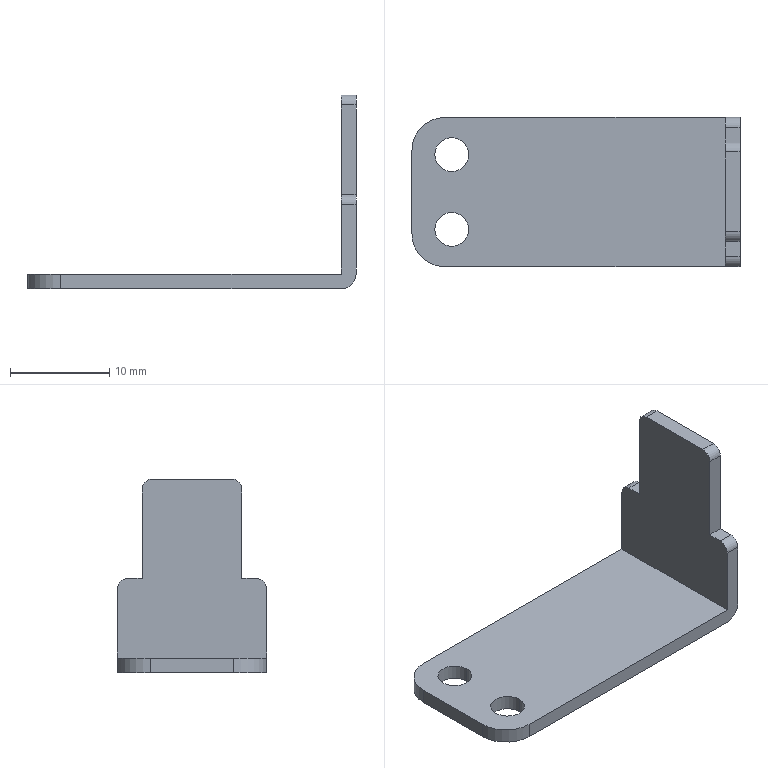Component | SolidWorks | V1ZHXTRR60SecondarySB1-1_V1ZHXT3.60InductionPlateSB1-1 | 1 solid | 23 faces | box 33 x 15 x 19.5 mm | volume 1030 mm3 | plane 12 | cylinder 11 | commonest cylinder face diameters 3.4 x4 2 x4 6.6 x2 3 x1
STEP:
#1=COLOUR_RGB('',0.7922,0.8196,0.9333);
#2=FILL_AREA_STYLE_COLOUR('',#1);
#3=FILL_AREA_STYLE('',(#2));
#4=SURFACE_STYLE_FILL_AREA(#3);
#5=SURFACE_SIDE_STYLE('',(#4));
#6=SURFACE_STYLE_USAGE(.BOTH.,#5);
#7=PRESENTATION_STYLE_ASSIGNMENT((#6));
#8=CARTESIAN_POINT('',(8.729,-7.889,17.903));
#9=VERTEX_POINT('',#8);
#10=CARTESIAN_POINT('',(8.595,-7.889,17.903));
#11=VERTEX_POINT('',#10);
#12=CARTESIAN_POINT('',(8.662,-7.889,17.903));
#13=DIRECTION('',(0.,-0.,1.));
#14=DIRECTION('',(1.,0.,0.));
#15=AXIS2_PLACEMENT_3D('',#12,#13,#14);
#16=CIRCLE('',#15,0.06693);
#17=EDGE_CURVE('',#9,#11,#16,.T.);
#18=ORIENTED_EDGE('',*,*,#17,.T.);
#19=CARTESIAN_POINT('',(8.595,-7.889,17.844));
#20=VERTEX_POINT('',#19);
#21=CARTESIAN_POINT('',(8.595,-7.889,17.844));
#22=DIRECTION('',(-0.,0.,-1.));
#23=VECTOR('',#22,39.37);
#24=LINE('',#21,#23);
#25=EDGE_CURVE('',#11,#20,#24,.T.);
#26=ORIENTED_EDGE('',*,*,#25,.T.);
#27=CARTESIAN_POINT('',(8.729,-7.889,17.844));
#28=VERTEX_POINT('',#27);
#29=CARTESIAN_POINT('',(8.662,-7.889,17.844));
#30=DIRECTION('',(0.,-0.,1.));
#31=DIRECTION('',(1.,0.,0.));
#32=AXIS2_PLACEMENT_3D('',#29,#30,#31);
#33=CIRCLE('',#32,0.06693);
#34=EDGE_CURVE('',#28,#20,#33,.T.);
#35=ORIENTED_EDGE('',*,*,#34,.F.);
#36=CARTESIAN_POINT('',(8.729,-7.889,17.844));
#37=DIRECTION('',(-0.,0.,-1.));
#38=VECTOR('',#37,39.37);
#39=LINE('',#36,#38);
#40=EDGE_CURVE('',#9,#28,#39,.T.);
#41=ORIENTED_EDGE('',*,*,#40,.F.);
#42=EDGE_LOOP('',(#18,#26,#35,#41));
#43=FACE_OUTER_BOUND('',#42,.T.);
#44=CARTESIAN_POINT('',(8.662,-7.889,17.844));
#45=DIRECTION('',(-0.,0.,-1.));
#46=DIRECTION('',(1.,0.,0.));
#47=AXIS2_PLACEMENT_3D('',#44,#45,#46);
#48=CYLINDRICAL_SURFACE('',#47,0.06693);
#49=ADVANCED_FACE('',(#43),#48,.F.);
#50=CARTESIAN_POINT('',(8.729,-8.184,17.903));
#51=VERTEX_POINT('',#50);
#52=CARTESIAN_POINT('',(8.595,-8.184,17.903));
#53=VERTEX_POINT('',#52);
#54=CARTESIAN_POINT('',(8.662,-8.184,17.903));
#55=DIRECTION('',(0.,-0.,1.));
#56=DIRECTION('',(1.,0.,0.));
#57=AXIS2_PLACEMENT_3D('',#54,#55,#56);
#58=CIRCLE('',#57,0.06693);
#59=EDGE_CURVE('',#51,#53,#58,.T.);
#60=ORIENTED_EDGE('',*,*,#59,.T.);
#61=CARTESIAN_POINT('',(8.595,-8.184,17.844));
#62=VERTEX_POINT('',#61);
#63=CARTESIAN_POINT('',(8.595,-8.184,17.844));
#64=DIRECTION('',(-0.,0.,-1.));
#65=VECTOR('',#64,39.37);
#66=LINE('',#63,#65);
#67=EDGE_CURVE('',#53,#62,#66,.T.);
#68=ORIENTED_EDGE('',*,*,#67,.T.);
#69=CARTESIAN_POINT('',(8.729,-8.184,17.844));
#70=VERTEX_POINT('',#69);
#71=CARTESIAN_POINT('',(8.662,-8.184,17.844));
#72=DIRECTION('',(0.,-0.,1.));
#73=DIRECTION('',(1.,0.,0.));
#74=AXIS2_PLACEMENT_3D('',#71,#72,#73);
#75=CIRCLE('',#74,0.06693);
#76=EDGE_CURVE('',#70,#62,#75,.T.);
#77=ORIENTED_EDGE('',*,*,#76,.F.);
#78=CARTESIAN_POINT('',(8.729,-8.184,17.844));
#79=DIRECTION('',(-0.,0.,-1.));
#80=VECTOR('',#79,39.37);
#81=LINE('',#78,#80);
#82=EDGE_CURVE('',#51,#70,#81,.T.);
#83=ORIENTED_EDGE('',*,*,#82,.F.);
#84=EDGE_LOOP('',(#60,#68,#77,#83));
#85=FACE_OUTER_BOUND('',#84,.T.);
#86=CARTESIAN_POINT('',(8.662,-8.184,17.844));
#87=DIRECTION('',(-0.,0.,-1.));
#88=DIRECTION('',(1.,0.,0.));
#89=AXIS2_PLACEMENT_3D('',#86,#87,#88);
#90=CYLINDRICAL_SURFACE('',#89,0.06693);
#91=ADVANCED_FACE('',(#85),#90,.F.);
#92=CARTESIAN_POINT('',(8.505,-7.871,17.903));
#93=VERTEX_POINT('',#92);
#94=CARTESIAN_POINT('',(8.635,-7.741,17.903));
#95=VERTEX_POINT('',#94);
#96=CARTESIAN_POINT('',(8.635,-7.871,17.903));
#97=DIRECTION('',(-0.,0.,-1.));
#98=DIRECTION('',(1.,0.,0.));
#99=AXIS2_PLACEMENT_3D('',#96,#97,#98);
#100=CIRCLE('',#99,0.1299);
#101=EDGE_CURVE('',#93,#95,#100,.T.);
#102=ORIENTED_EDGE('',*,*,#101,.F.);
#103=CARTESIAN_POINT('',(8.505,-8.202,17.903));
#104=VERTEX_POINT('',#103);
#105=CARTESIAN_POINT('',(8.505,-8.332,17.903));
#106=DIRECTION('',(-0.,1.,0.));
#107=VECTOR('',#106,39.37);
#108=LINE('',#105,#107);
#109=EDGE_CURVE('',#104,#93,#108,.T.);
#110=ORIENTED_EDGE('',*,*,#109,.F.);
#111=CARTESIAN_POINT('',(8.635,-8.332,17.903));
#112=VERTEX_POINT('',#111);
#113=CARTESIAN_POINT('',(8.635,-8.202,17.903));
#114=DIRECTION('',(-0.,0.,-1.));
#115=DIRECTION('',(1.,0.,0.));
#116=AXIS2_PLACEMENT_3D('',#113,#114,#115);
#117=CIRCLE('',#116,0.1299);
#118=EDGE_CURVE('',#112,#104,#117,.T.);
#119=ORIENTED_EDGE('',*,*,#118,.F.);
#120=CARTESIAN_POINT('',(9.745,-8.332,17.903));
#121=VERTEX_POINT('',#120);
#122=CARTESIAN_POINT('',(9.804,-8.332,17.903));
#123=DIRECTION('',(-1.,-0.,0.));
#124=VECTOR('',#123,39.37);
#125=LINE('',#122,#124);
#126=EDGE_CURVE('',#121,#112,#125,.T.);
#127=ORIENTED_EDGE('',*,*,#126,.F.);
#128=CARTESIAN_POINT('',(9.745,-7.741,17.903));
#129=VERTEX_POINT('',#128);
#130=CARTESIAN_POINT('',(9.745,-8.332,17.903));
#131=DIRECTION('',(0.,-1.,-0.));
#132=VECTOR('',#131,39.37);
#133=LINE('',#130,#132);
#134=EDGE_CURVE('',#129,#121,#133,.T.);
#135=ORIENTED_EDGE('',*,*,#134,.F.);
#136=CARTESIAN_POINT('',(9.804,-7.741,17.903));
#137=DIRECTION('',(1.,0.,-0.));
#138=VECTOR('',#137,39.37);
#139=LINE('',#136,#138);
#140=EDGE_CURVE('',#95,#129,#139,.T.);
#141=ORIENTED_EDGE('',*,*,#140,.F.);
#142=EDGE_LOOP('',(#102,#110,#119,#127,#135,#141));
#143=FACE_OUTER_BOUND('',#142,.T.);
#144=ORIENTED_EDGE('',*,*,#17,.F.);
#145=CARTESIAN_POINT('',(8.662,-7.889,17.903));
#146=DIRECTION('',(0.,-0.,1.));
#147=DIRECTION('',(1.,0.,0.));
#148=AXIS2_PLACEMENT_3D('',#145,#146,#147);
#149=CIRCLE('',#148,0.06693);
#150=EDGE_CURVE('',#11,#9,#149,.T.);
#151=ORIENTED_EDGE('',*,*,#150,.F.);
#152=EDGE_LOOP('',(#144,#151));
#153=FACE_BOUND('',#152,.T.);
#154=ORIENTED_EDGE('',*,*,#59,.F.);
#155=CARTESIAN_POINT('',(8.662,-8.184,17.903));
#156=DIRECTION('',(0.,-0.,1.));
#157=DIRECTION('',(1.,0.,0.));
#158=AXIS2_PLACEMENT_3D('',#155,#156,#157);
#159=CIRCLE('',#158,0.06693);
#160=EDGE_CURVE('',#53,#51,#159,.T.);
#161=ORIENTED_EDGE('',*,*,#160,.F.);
#162=EDGE_LOOP('',(#154,#161));
#163=FACE_BOUND('',#162,.T.);
#164=CARTESIAN_POINT('',(9.804,-8.332,17.903));
#165=DIRECTION('',(-0.,0.,-1.));
#166=DIRECTION('',(1.,0.,-0.));
#167=AXIS2_PLACEMENT_3D('',#164,#165,#166);
#168=PLANE('',#167);
#169=ADVANCED_FACE('',(#143,#153,#163),#168,.F.);
#170=CARTESIAN_POINT('',(9.745,-7.741,17.844));
#171=VERTEX_POINT('',#170);
#172=CARTESIAN_POINT('',(9.804,-7.741,17.903));
#173=VERTEX_POINT('',#172);
#174=CARTESIAN_POINT('',(9.745,-7.741,17.903));
#175=DIRECTION('',(0.,-1.,-0.));
#176=DIRECTION('',(0.,-0.,1.));
#177=AXIS2_PLACEMENT_3D('',#174,#175,#176);
#178=CIRCLE('',#177,0.05906);
#179=EDGE_CURVE('',#171,#173,#178,.T.);
#180=ORIENTED_EDGE('',*,*,#179,.F.);
#181=CARTESIAN_POINT('',(8.635,-7.741,17.844));
#182=VERTEX_POINT('',#181);
#183=CARTESIAN_POINT('',(9.804,-7.741,17.844));
#184=DIRECTION('',(1.,0.,-0.));
#185=VECTOR('',#184,39.37);
#186=LINE('',#183,#185);
#187=EDGE_CURVE('',#182,#171,#186,.T.);
#188=ORIENTED_EDGE('',*,*,#187,.F.);
#189=CARTESIAN_POINT('',(8.635,-7.741,17.903));
#190=DIRECTION('',(-0.,0.,-1.));
#191=VECTOR('',#190,39.37);
#192=LINE('',#189,#191);
#193=EDGE_CURVE('',#95,#182,#192,.T.);
#194=ORIENTED_EDGE('',*,*,#193,.F.);
#195=ORIENTED_EDGE('',*,*,#140,.T.);
#196=CARTESIAN_POINT('',(9.745,-7.741,18.179));
#197=VERTEX_POINT('',#196);
#198=CARTESIAN_POINT('',(9.745,-7.741,17.903));
#199=DIRECTION('',(-0.,0.,-1.));
#200=VECTOR('',#199,39.37);
#201=LINE('',#198,#200);
#202=EDGE_CURVE('',#197,#129,#201,.T.);
#203=ORIENTED_EDGE('',*,*,#202,.F.);
#204=CARTESIAN_POINT('',(9.804,-7.741,18.179));
#205=VERTEX_POINT('',#204);
#206=CARTESIAN_POINT('',(9.804,-7.741,18.179));
#207=DIRECTION('',(-1.,-0.,0.));
#208=VECTOR('',#207,39.37);
#209=LINE('',#206,#208);
#210=EDGE_CURVE('',#205,#197,#209,.T.);
#211=ORIENTED_EDGE('',*,*,#210,.F.);
#212=CARTESIAN_POINT('',(9.804,-7.741,17.903));
#213=DIRECTION('',(0.,-0.,1.));
#214=VECTOR('',#213,39.37);
#215=LINE('',#212,#214);
#216=EDGE_CURVE('',#173,#205,#215,.T.);
#217=ORIENTED_EDGE('',*,*,#216,.F.);
#218=EDGE_LOOP('',(#180,#188,#194,#195,#203,#211,#217));
#219=FACE_OUTER_BOUND('',#218,.T.);
#220=CARTESIAN_POINT('',(9.804,-7.741,17.903));
#221=DIRECTION('',(0.,-1.,-0.));
#222=DIRECTION('',(0.,-0.,1.));
#223=AXIS2_PLACEMENT_3D('',#220,#221,#222);
#224=PLANE('',#223);
#225=ADVANCED_FACE('',(#219),#224,.F.);
#226=CARTESIAN_POINT('',(8.505,-7.871,17.844));
#227=VERTEX_POINT('',#226);
#228=CARTESIAN_POINT('',(8.635,-7.871,17.844));
#229=DIRECTION('',(0.,-0.,1.));
#230=DIRECTION('',(1.,0.,0.));
#231=AXIS2_PLACEMENT_3D('',#228,#229,#230);
#232=CIRCLE('',#231,0.1299);
#233=EDGE_CURVE('',#182,#227,#232,.T.);
#234=ORIENTED_EDGE('',*,*,#233,.T.);
#235=CARTESIAN_POINT('',(8.505,-7.871,17.903));
#236=DIRECTION('',(0.,-0.,1.));
#237=VECTOR('',#236,39.37);
#238=LINE('',#235,#237);
#239=EDGE_CURVE('',#227,#93,#238,.T.);
#240=ORIENTED_EDGE('',*,*,#239,.T.);
#241=ORIENTED_EDGE('',*,*,#101,.T.);
#242=ORIENTED_EDGE('',*,*,#193,.T.);
#243=EDGE_LOOP('',(#234,#240,#241,#242));
#244=FACE_OUTER_BOUND('',#243,.T.);
#245=CARTESIAN_POINT('',(8.635,-7.871,17.903));
#246=DIRECTION('',(-0.,0.,-1.));
#247=DIRECTION('',(1.,0.,0.));
#248=AXIS2_PLACEMENT_3D('',#245,#246,#247);
#249=CYLINDRICAL_SURFACE('',#248,0.1299);
#250=ADVANCED_FACE('',(#244),#249,.T.);
#251=ORIENTED_EDGE('',*,*,#239,.F.);
#252=CARTESIAN_POINT('',(8.505,-8.202,17.844));
#253=VERTEX_POINT('',#252);
#254=CARTESIAN_POINT('',(8.505,-7.741,17.844));
#255=DIRECTION('',(-0.,1.,0.));
#256=VECTOR('',#255,39.37);
#257=LINE('',#254,#256);
#258=EDGE_CURVE('',#253,#227,#257,.T.);
#259=ORIENTED_EDGE('',*,*,#258,.F.);
#260=CARTESIAN_POINT('',(8.505,-8.202,17.903));
#261=DIRECTION('',(-0.,0.,-1.));
#262=VECTOR('',#261,39.37);
#263=LINE('',#260,#262);
#264=EDGE_CURVE('',#104,#253,#263,.T.);
#265=ORIENTED_EDGE('',*,*,#264,.F.);
#266=ORIENTED_EDGE('',*,*,#109,.T.);
#267=EDGE_LOOP('',(#251,#259,#265,#266));
#268=FACE_OUTER_BOUND('',#267,.T.);
#269=CARTESIAN_POINT('',(8.505,-7.741,17.903));
#270=DIRECTION('',(1.,0.,-0.));
#271=DIRECTION('',(0.,-0.,1.));
#272=AXIS2_PLACEMENT_3D('',#269,#270,#271);
#273=PLANE('',#272);
#274=ADVANCED_FACE('',(#268),#273,.F.);
#275=CARTESIAN_POINT('',(8.635,-8.332,17.844));
#276=VERTEX_POINT('',#275);
#277=CARTESIAN_POINT('',(8.635,-8.202,17.844));
#278=DIRECTION('',(0.,-0.,1.));
#279=DIRECTION('',(1.,0.,0.));
#280=AXIS2_PLACEMENT_3D('',#277,#278,#279);
#281=CIRCLE('',#280,0.1299);
#282=EDGE_CURVE('',#253,#276,#281,.T.);
#283=ORIENTED_EDGE('',*,*,#282,.T.);
#284=CARTESIAN_POINT('',(8.635,-8.332,17.903));
#285=DIRECTION('',(0.,-0.,1.));
#286=VECTOR('',#285,39.37);
#287=LINE('',#284,#286);
#288=EDGE_CURVE('',#276,#112,#287,.T.);
#289=ORIENTED_EDGE('',*,*,#288,.T.);
#290=ORIENTED_EDGE('',*,*,#118,.T.);
#291=ORIENTED_EDGE('',*,*,#264,.T.);
#292=EDGE_LOOP('',(#283,#289,#290,#291));
#293=FACE_OUTER_BOUND('',#292,.T.);
#294=CARTESIAN_POINT('',(8.635,-8.202,17.903));
#295=DIRECTION('',(-0.,0.,-1.));
#296=DIRECTION('',(1.,0.,0.));
#297=AXIS2_PLACEMENT_3D('',#294,#295,#296);
#298=CYLINDRICAL_SURFACE('',#297,0.1299);
#299=ADVANCED_FACE('',(#293),#298,.T.);
#300=CARTESIAN_POINT('',(9.804,-8.332,17.903));
#301=VERTEX_POINT('',#300);
#302=CARTESIAN_POINT('',(9.745,-8.332,17.844));
#303=VERTEX_POINT('',#302);
#304=CARTESIAN_POINT('',(9.745,-8.332,17.903));
#305=DIRECTION('',(-0.,1.,0.));
#306=DIRECTION('',(0.,-0.,1.));
#307=AXIS2_PLACEMENT_3D('',#304,#305,#306);
#308=CIRCLE('',#307,0.05906);
#309=EDGE_CURVE('',#301,#303,#308,.T.);
#310=ORIENTED_EDGE('',*,*,#309,.F.);
#311=CARTESIAN_POINT('',(9.804,-8.332,18.179));
#312=VERTEX_POINT('',#311);
#313=CARTESIAN_POINT('',(9.804,-8.332,17.903));
#314=DIRECTION('',(-0.,0.,-1.));
#315=VECTOR('',#314,39.37);
#316=LINE('',#313,#315);
#317=EDGE_CURVE('',#312,#301,#316,.T.);
#318=ORIENTED_EDGE('',*,*,#317,.F.);
#319=CARTESIAN_POINT('',(9.745,-8.332,18.179));
#320=VERTEX_POINT('',#319);
#321=CARTESIAN_POINT('',(9.804,-8.332,18.179));
#322=DIRECTION('',(1.,0.,-0.));
#323=VECTOR('',#322,39.37);
#324=LINE('',#321,#323);
#325=EDGE_CURVE('',#320,#312,#324,.T.);
#326=ORIENTED_EDGE('',*,*,#325,.F.);
#327=CARTESIAN_POINT('',(9.745,-8.332,17.903));
#328=DIRECTION('',(0.,-0.,1.));
#329=VECTOR('',#328,39.37);
#330=LINE('',#327,#329);
#331=EDGE_CURVE('',#121,#320,#330,.T.);
#332=ORIENTED_EDGE('',*,*,#331,.F.);
#333=ORIENTED_EDGE('',*,*,#126,.T.);
#334=ORIENTED_EDGE('',*,*,#288,.F.);
#335=CARTESIAN_POINT('',(9.804,-8.332,17.844));
#336=DIRECTION('',(-1.,-0.,0.));
#337=VECTOR('',#336,39.37);
#338=LINE('',#335,#337);
#339=EDGE_CURVE('',#303,#276,#338,.T.);
#340=ORIENTED_EDGE('',*,*,#339,.F.);
#341=EDGE_LOOP('',(#310,#318,#326,#332,#333,#334,#340));
#342=FACE_OUTER_BOUND('',#341,.T.);
#343=CARTESIAN_POINT('',(9.804,-8.332,17.903));
#344=DIRECTION('',(-0.,1.,0.));
#345=DIRECTION('',(-0.,0.,-1.));
#346=AXIS2_PLACEMENT_3D('',#343,#344,#345);
#347=PLANE('',#346);
#348=ADVANCED_FACE('',(#342),#347,.F.);
#349=CARTESIAN_POINT('',(9.745,-8.293,18.218));
#350=VERTEX_POINT('',#349);
#351=CARTESIAN_POINT('',(9.745,-8.293,18.179));
#352=DIRECTION('',(1.,0.,-0.));
#353=DIRECTION('',(0.,-0.,1.));
#354=AXIS2_PLACEMENT_3D('',#351,#352,#353);
#355=CIRCLE('',#354,0.03937);
#356=EDGE_CURVE('',#350,#320,#355,.T.);
#357=ORIENTED_EDGE('',*,*,#356,.F.);
#358=CARTESIAN_POINT('',(9.745,-8.234,18.218));
#359=VERTEX_POINT('',#358);
#360=CARTESIAN_POINT('',(9.745,-8.332,18.218));
#361=DIRECTION('',(0.,-1.,-0.));
#362=VECTOR('',#361,39.37);
#363=LINE('',#360,#362);
#364=EDGE_CURVE('',#359,#350,#363,.T.);
#365=ORIENTED_EDGE('',*,*,#364,.F.);
#366=CARTESIAN_POINT('',(9.745,-8.234,18.572));
#367=VERTEX_POINT('',#366);
#368=CARTESIAN_POINT('',(9.745,-8.234,18.612));
#369=DIRECTION('',(-0.,0.,-1.));
#370=VECTOR('',#369,39.37);
#371=LINE('',#368,#370);
#372=EDGE_CURVE('',#367,#359,#371,.T.);
#373=ORIENTED_EDGE('',*,*,#372,.F.);
#374=CARTESIAN_POINT('',(9.745,-8.194,18.612));
#375=VERTEX_POINT('',#374);
#376=CARTESIAN_POINT('',(9.745,-8.194,18.572));
#377=DIRECTION('',(1.,0.,-0.));
#378=DIRECTION('',(0.,-0.,1.));
#379=AXIS2_PLACEMENT_3D('',#376,#377,#378);
#380=CIRCLE('',#379,0.03937);
#381=EDGE_CURVE('',#375,#367,#380,.T.);
#382=ORIENTED_EDGE('',*,*,#381,.F.);
#383=CARTESIAN_POINT('',(9.745,-7.879,18.612));
#384=VERTEX_POINT('',#383);
#385=CARTESIAN_POINT('',(9.745,-8.332,18.612));
#386=DIRECTION('',(0.,-1.,-0.));
#387=VECTOR('',#386,39.37);
#388=LINE('',#385,#387);
#389=EDGE_CURVE('',#384,#375,#388,.T.);
#390=ORIENTED_EDGE('',*,*,#389,.F.);
#391=CARTESIAN_POINT('',(9.745,-7.84,18.572));
#392=VERTEX_POINT('',#391);
#393=CARTESIAN_POINT('',(9.745,-7.879,18.572));
#394=DIRECTION('',(1.,0.,-0.));
#395=DIRECTION('',(0.,0.,-1.));
#396=AXIS2_PLACEMENT_3D('',#393,#394,#395);
#397=CIRCLE('',#396,0.03937);
#398=EDGE_CURVE('',#392,#384,#397,.T.);
#399=ORIENTED_EDGE('',*,*,#398,.F.);
#400=CARTESIAN_POINT('',(9.745,-7.84,18.218));
#401=VERTEX_POINT('',#400);
#402=CARTESIAN_POINT('',(9.745,-7.84,18.612));
#403=DIRECTION('',(0.,-0.,1.));
#404=VECTOR('',#403,39.37);
#405=LINE('',#402,#404);
#406=EDGE_CURVE('',#401,#392,#405,.T.);
#407=ORIENTED_EDGE('',*,*,#406,.F.);
#408=CARTESIAN_POINT('',(9.745,-7.781,18.218));
#409=VERTEX_POINT('',#408);
#410=CARTESIAN_POINT('',(9.745,-8.332,18.218));
#411=DIRECTION('',(0.,-1.,-0.));
#412=VECTOR('',#411,39.37);
#413=LINE('',#410,#412);
#414=EDGE_CURVE('',#409,#401,#413,.T.);
#415=ORIENTED_EDGE('',*,*,#414,.F.);
#416=CARTESIAN_POINT('',(9.745,-7.781,18.179));
#417=DIRECTION('',(1.,0.,-0.));
#418=DIRECTION('',(0.,-0.,1.));
#419=AXIS2_PLACEMENT_3D('',#416,#417,#418);
#420=CIRCLE('',#419,0.03937);
#421=EDGE_CURVE('',#197,#409,#420,.T.);
#422=ORIENTED_EDGE('',*,*,#421,.F.);
#423=ORIENTED_EDGE('',*,*,#202,.T.);
#424=ORIENTED_EDGE('',*,*,#134,.T.);
#425=ORIENTED_EDGE('',*,*,#331,.T.);
#426=EDGE_LOOP('',(#357,#365,#373,#382,#390,#399,#407,#415,#422,#423,#424,#425));
#427=FACE_OUTER_BOUND('',#426,.T.);
#428=CARTESIAN_POINT('',(9.745,-8.332,18.612));
#429=DIRECTION('',(1.,0.,-0.));
#430=DIRECTION('',(-0.,1.,0.));
#431=AXIS2_PLACEMENT_3D('',#428,#429,#430);
#432=PLANE('',#431);
#433=ADVANCED_FACE('',(#427),#432,.F.);
#434=ORIENTED_EDGE('',*,*,#25,.F.);
#435=ORIENTED_EDGE('',*,*,#150,.T.);
#436=ORIENTED_EDGE('',*,*,#40,.T.);
#437=CARTESIAN_POINT('',(8.662,-7.889,17.844));
#438=DIRECTION('',(0.,-0.,1.));
#439=DIRECTION('',(1.,0.,0.));
#440=AXIS2_PLACEMENT_3D('',#437,#438,#439);
#441=CIRCLE('',#440,0.06693);
#442=EDGE_CURVE('',#20,#28,#441,.T.);
#443=ORIENTED_EDGE('',*,*,#442,.F.);
#444=EDGE_LOOP('',(#434,#435,#436,#443));
#445=FACE_OUTER_BOUND('',#444,.T.);
#446=CARTESIAN_POINT('',(8.662,-7.889,17.844));
#447=DIRECTION('',(-0.,0.,-1.));
#448=DIRECTION('',(1.,0.,0.));
#449=AXIS2_PLACEMENT_3D('',#446,#447,#448);
#450=CYLINDRICAL_SURFACE('',#449,0.06693);
#451=ADVANCED_FACE('',(#445),#450,.F.);
#452=ORIENTED_EDGE('',*,*,#67,.F.);
#453=ORIENTED_EDGE('',*,*,#160,.T.);
#454=ORIENTED_EDGE('',*,*,#82,.T.);
#455=CARTESIAN_POINT('',(8.662,-8.184,17.844));
#456=DIRECTION('',(0.,-0.,1.));
#457=DIRECTION('',(1.,0.,0.));
#458=AXIS2_PLACEMENT_3D('',#455,#456,#457);
#459=CIRCLE('',#458,0.06693);
#460=EDGE_CURVE('',#62,#70,#459,.T.);
#461=ORIENTED_EDGE('',*,*,#460,.F.);
#462=EDGE_LOOP('',(#452,#453,#454,#461));
#463=FACE_OUTER_BOUND('',#462,.T.);
#464=CARTESIAN_POINT('',(8.662,-8.184,17.844));
#465=DIRECTION('',(-0.,0.,-1.));
#466=DIRECTION('',(1.,0.,0.));
#467=AXIS2_PLACEMENT_3D('',#464,#465,#466);
#468=CYLINDRICAL_SURFACE('',#467,0.06693);
#469=ADVANCED_FACE('',(#463),#468,.F.);
#470=CARTESIAN_POINT('',(9.804,-7.741,17.903));
#471=DIRECTION('',(0.,-1.,-0.));
#472=VECTOR('',#471,39.37);
#473=LINE('',#470,#472);
#474=EDGE_CURVE('',#173,#301,#473,.T.);
#475=ORIENTED_EDGE('',*,*,#474,.F.);
#476=ORIENTED_EDGE('',*,*,#216,.T.);
#477=CARTESIAN_POINT('',(9.804,-7.781,18.218));
#478=VERTEX_POINT('',#477);
#479=CARTESIAN_POINT('',(9.804,-7.781,18.179));
#480=DIRECTION('',(-1.,-0.,0.));
#481=DIRECTION('',(0.,-0.,1.));
#482=AXIS2_PLACEMENT_3D('',#479,#480,#481);
#483=CIRCLE('',#482,0.03937);
#484=EDGE_CURVE('',#478,#205,#483,.T.);
#485=ORIENTED_EDGE('',*,*,#484,.F.);
#486=CARTESIAN_POINT('',(9.804,-7.84,18.218));
#487=VERTEX_POINT('',#486);
#488=CARTESIAN_POINT('',(9.804,-7.741,18.218));
#489=DIRECTION('',(-0.,1.,0.));
#490=VECTOR('',#489,39.37);
#491=LINE('',#488,#490);
#492=EDGE_CURVE('',#487,#478,#491,.T.);
#493=ORIENTED_EDGE('',*,*,#492,.F.);
#494=CARTESIAN_POINT('',(9.804,-7.84,18.572));
#495=VERTEX_POINT('',#494);
#496=CARTESIAN_POINT('',(9.804,-7.84,17.903));
#497=DIRECTION('',(-0.,0.,-1.));
#498=VECTOR('',#497,39.37);
#499=LINE('',#496,#498);
#500=EDGE_CURVE('',#495,#487,#499,.T.);
#501=ORIENTED_EDGE('',*,*,#500,.F.);
#502=CARTESIAN_POINT('',(9.804,-7.879,18.612));
#503=VERTEX_POINT('',#502);
#504=CARTESIAN_POINT('',(9.804,-7.879,18.572));
#505=DIRECTION('',(-1.,-0.,0.));
#506=DIRECTION('',(0.,0.,-1.));
#507=AXIS2_PLACEMENT_3D('',#504,#505,#506);
#508=CIRCLE('',#507,0.03937);
#509=EDGE_CURVE('',#503,#495,#508,.T.);
#510=ORIENTED_EDGE('',*,*,#509,.F.);
#511=CARTESIAN_POINT('',(9.804,-8.194,18.612));
#512=VERTEX_POINT('',#511);
#513=CARTESIAN_POINT('',(9.804,-7.741,18.612));
#514=DIRECTION('',(-0.,1.,0.));
#515=VECTOR('',#514,39.37);
#516=LINE('',#513,#515);
#517=EDGE_CURVE('',#512,#503,#516,.T.);
#518=ORIENTED_EDGE('',*,*,#517,.F.);
#519=CARTESIAN_POINT('',(9.804,-8.234,18.572));
#520=VERTEX_POINT('',#519);
#521=CARTESIAN_POINT('',(9.804,-8.194,18.572));
#522=DIRECTION('',(-1.,-0.,0.));
#523=DIRECTION('',(0.,-0.,1.));
#524=AXIS2_PLACEMENT_3D('',#521,#522,#523);
#525=CIRCLE('',#524,0.03937);
#526=EDGE_CURVE('',#520,#512,#525,.T.);
#527=ORIENTED_EDGE('',*,*,#526,.F.);
#528=CARTESIAN_POINT('',(9.804,-8.234,18.218));
#529=VERTEX_POINT('',#528);
#530=CARTESIAN_POINT('',(9.804,-8.234,17.903));
#531=DIRECTION('',(0.,-0.,1.));
#532=VECTOR('',#531,39.37);
#533=LINE('',#530,#532);
#534=EDGE_CURVE('',#529,#520,#533,.T.);
#535=ORIENTED_EDGE('',*,*,#534,.F.);
#536=CARTESIAN_POINT('',(9.804,-8.293,18.218));
#537=VERTEX_POINT('',#536);
#538=CARTESIAN_POINT('',(9.804,-7.741,18.218));
#539=DIRECTION('',(-0.,1.,0.));
#540=VECTOR('',#539,39.37);
#541=LINE('',#538,#540);
#542=EDGE_CURVE('',#537,#529,#541,.T.);
#543=ORIENTED_EDGE('',*,*,#542,.F.);
#544=CARTESIAN_POINT('',(9.804,-8.293,18.179));
#545=DIRECTION('',(-1.,-0.,0.));
#546=DIRECTION('',(0.,-0.,1.));
#547=AXIS2_PLACEMENT_3D('',#544,#545,#546);
#548=CIRCLE('',#547,0.03937);
#549=EDGE_CURVE('',#312,#537,#548,.T.);
#550=ORIENTED_EDGE('',*,*,#549,.F.);
#551=ORIENTED_EDGE('',*,*,#317,.T.);
#552=EDGE_LOOP('',(#475,#476,#485,#493,#501,#510,#518,#527,#535,#543,#550,#551));
#553=FACE_OUTER_BOUND('',#552,.T.);
#554=CARTESIAN_POINT('',(9.804,-7.741,17.903));
#555=DIRECTION('',(-1.,-0.,0.));
#556=DIRECTION('',(-0.,0.,-1.));
#557=AXIS2_PLACEMENT_3D('',#554,#555,#556);
#558=PLANE('',#557);
#559=ADVANCED_FACE('',(#553),#558,.F.);
#560=ORIENTED_EDGE('',*,*,#179,.T.);
#561=ORIENTED_EDGE('',*,*,#474,.T.);
#562=ORIENTED_EDGE('',*,*,#309,.T.);
#563=CARTESIAN_POINT('',(9.745,-7.741,17.844));
#564=DIRECTION('',(-0.,1.,0.));
#565=VECTOR('',#564,39.37);
#566=LINE('',#563,#565);
#567=EDGE_CURVE('',#303,#171,#566,.T.);
#568=ORIENTED_EDGE('',*,*,#567,.T.);
#569=EDGE_LOOP('',(#560,#561,#562,#568));
#570=FACE_OUTER_BOUND('',#569,.T.);
#571=CARTESIAN_POINT('',(9.745,-7.741,17.903));
#572=DIRECTION('',(0.,-1.,-0.));
#573=DIRECTION('',(0.,-0.,1.));
#574=AXIS2_PLACEMENT_3D('',#571,#572,#573);
#575=CYLINDRICAL_SURFACE('',#574,0.05906);
#576=ADVANCED_FACE('',(#570),#575,.T.);
#577=ORIENTED_EDGE('',*,*,#258,.T.);
#578=ORIENTED_EDGE('',*,*,#233,.F.);
#579=ORIENTED_EDGE('',*,*,#187,.T.);
#580=ORIENTED_EDGE('',*,*,#567,.F.);
#581=ORIENTED_EDGE('',*,*,#339,.T.);
#582=ORIENTED_EDGE('',*,*,#282,.F.);
#583=EDGE_LOOP('',(#577,#578,#579,#580,#581,#582));
#584=FACE_OUTER_BOUND('',#583,.T.);
#585=ORIENTED_EDGE('',*,*,#34,.T.);
#586=ORIENTED_EDGE('',*,*,#442,.T.);
#587=EDGE_LOOP('',(#585,#586));
#588=FACE_BOUND('',#587,.T.);
#589=ORIENTED_EDGE('',*,*,#76,.T.);
#590=ORIENTED_EDGE('',*,*,#460,.T.);
#591=EDGE_LOOP('',(#589,#590));
#592=FACE_BOUND('',#591,.T.);
#593=CARTESIAN_POINT('',(9.804,-8.332,17.844));
#594=DIRECTION('',(-0.,0.,-1.));
#595=DIRECTION('',(1.,0.,-0.));
#596=AXIS2_PLACEMENT_3D('',#593,#594,#595);
#597=PLANE('',#596);
#598=ADVANCED_FACE('',(#584,#588,#592),#597,.T.);
#599=ORIENTED_EDGE('',*,*,#484,.T.);
#600=ORIENTED_EDGE('',*,*,#210,.T.);
#601=ORIENTED_EDGE('',*,*,#421,.T.);
#602=CARTESIAN_POINT('',(9.804,-7.781,18.218));
#603=DIRECTION('',(1.,0.,-0.));
#604=VECTOR('',#603,39.37);
#605=LINE('',#602,#604);
#606=EDGE_CURVE('',#409,#478,#605,.T.);
#607=ORIENTED_EDGE('',*,*,#606,.T.);
#608=EDGE_LOOP('',(#599,#600,#601,#607));
#609=FACE_OUTER_BOUND('',#608,.T.);
#610=CARTESIAN_POINT('',(9.804,-7.781,18.179));
#611=DIRECTION('',(1.,0.,-0.));
#612=DIRECTION('',(0.,-0.,1.));
#613=AXIS2_PLACEMENT_3D('',#610,#611,#612);
#614=CYLINDRICAL_SURFACE('',#613,0.03937);
#615=ADVANCED_FACE('',(#609),#614,.T.);
#616=ORIENTED_EDGE('',*,*,#549,.T.);
#617=CARTESIAN_POINT('',(8.505,-8.293,18.218));
#618=DIRECTION('',(-1.,-0.,0.));
#619=VECTOR('',#618,39.37);
#620=LINE('',#617,#619);
#621=EDGE_CURVE('',#537,#350,#620,.T.);
#622=ORIENTED_EDGE('',*,*,#621,.T.);
#623=ORIENTED_EDGE('',*,*,#356,.T.);
#624=ORIENTED_EDGE('',*,*,#325,.T.);
#625=EDGE_LOOP('',(#616,#622,#623,#624));
#626=FACE_OUTER_BOUND('',#625,.T.);
#627=CARTESIAN_POINT('',(8.505,-8.293,18.179));
#628=DIRECTION('',(1.,0.,-0.));
#629=DIRECTION('',(0.,-0.,1.));
#630=AXIS2_PLACEMENT_3D('',#627,#628,#629);
#631=CYLINDRICAL_SURFACE('',#630,0.03937);
#632=ADVANCED_FACE('',(#626),#631,.T.);
#633=ORIENTED_EDGE('',*,*,#621,.F.);
#634=ORIENTED_EDGE('',*,*,#542,.T.);
#635=CARTESIAN_POINT('',(8.505,-8.234,18.218));
#636=DIRECTION('',(1.,0.,-0.));
#637=VECTOR('',#636,39.37);
#638=LINE('',#635,#637);
#639=EDGE_CURVE('',#359,#529,#638,.T.);
#640=ORIENTED_EDGE('',*,*,#639,.F.);
#641=ORIENTED_EDGE('',*,*,#364,.T.);
#642=EDGE_LOOP('',(#633,#634,#640,#641));
#643=FACE_OUTER_BOUND('',#642,.T.);
#644=CARTESIAN_POINT('',(8.505,-8.332,18.218));
#645=DIRECTION('',(-0.,0.,-1.));
#646=DIRECTION('',(1.,0.,-0.));
#647=AXIS2_PLACEMENT_3D('',#644,#645,#646);
#648=PLANE('',#647);
#649=ADVANCED_FACE('',(#643),#648,.F.);
#650=CARTESIAN_POINT('',(8.505,-8.234,18.572));
#651=DIRECTION('',(1.,0.,-0.));
#652=VECTOR('',#651,39.37);
#653=LINE('',#650,#652);
#654=EDGE_CURVE('',#367,#520,#653,.T.);
#655=ORIENTED_EDGE('',*,*,#654,.F.);
#656=ORIENTED_EDGE('',*,*,#372,.T.);
#657=ORIENTED_EDGE('',*,*,#639,.T.);
#658=ORIENTED_EDGE('',*,*,#534,.T.);
#659=EDGE_LOOP('',(#655,#656,#657,#658));
#660=FACE_OUTER_BOUND('',#659,.T.);
#661=CARTESIAN_POINT('',(8.505,-8.234,18.612));
#662=DIRECTION('',(-0.,1.,0.));
#663=DIRECTION('',(-0.,0.,-1.));
#664=AXIS2_PLACEMENT_3D('',#661,#662,#663);
#665=PLANE('',#664);
#666=ADVANCED_FACE('',(#660),#665,.F.);
#667=ORIENTED_EDGE('',*,*,#381,.T.);
#668=ORIENTED_EDGE('',*,*,#654,.T.);
#669=ORIENTED_EDGE('',*,*,#526,.T.);
#670=CARTESIAN_POINT('',(8.505,-8.194,18.612));
#671=DIRECTION('',(-1.,-0.,0.));
#672=VECTOR('',#671,39.37);
#673=LINE('',#670,#672);
#674=EDGE_CURVE('',#512,#375,#673,.T.);
#675=ORIENTED_EDGE('',*,*,#674,.T.);
#676=EDGE_LOOP('',(#667,#668,#669,#675));
#677=FACE_OUTER_BOUND('',#676,.T.);
#678=CARTESIAN_POINT('',(8.505,-8.194,18.572));
#679=DIRECTION('',(1.,0.,-0.));
#680=DIRECTION('',(0.,-0.,1.));
#681=AXIS2_PLACEMENT_3D('',#678,#679,#680);
#682=CYLINDRICAL_SURFACE('',#681,0.03937);
#683=ADVANCED_FACE('',(#677),#682,.T.);
#684=ORIENTED_EDGE('',*,*,#389,.T.);
#685=ORIENTED_EDGE('',*,*,#674,.F.);
#686=ORIENTED_EDGE('',*,*,#517,.T.);
#687=CARTESIAN_POINT('',(9.804,-7.879,18.612));
#688=DIRECTION('',(-1.,-0.,0.));
#689=VECTOR('',#688,39.37);
#690=LINE('',#687,#689);
#691=EDGE_CURVE('',#503,#384,#690,.T.);
#692=ORIENTED_EDGE('',*,*,#691,.T.);
#693=EDGE_LOOP('',(#684,#685,#686,#692));
#694=FACE_OUTER_BOUND('',#693,.T.);
#695=CARTESIAN_POINT('',(9.804,-7.741,18.612));
#696=DIRECTION('',(0.,-0.,1.));
#697=DIRECTION('',(-1.,-0.,0.));
#698=AXIS2_PLACEMENT_3D('',#695,#696,#697);
#699=PLANE('',#698);
#700=ADVANCED_FACE('',(#694),#699,.T.);
#701=ORIENTED_EDGE('',*,*,#509,.T.);
#702=CARTESIAN_POINT('',(8.505,-7.84,18.572));
#703=DIRECTION('',(-1.,-0.,0.));
#704=VECTOR('',#703,39.37);
#705=LINE('',#702,#704);
#706=EDGE_CURVE('',#495,#392,#705,.T.);
#707=ORIENTED_EDGE('',*,*,#706,.T.);
#708=ORIENTED_EDGE('',*,*,#398,.T.);
#709=ORIENTED_EDGE('',*,*,#691,.F.);
#710=EDGE_LOOP('',(#701,#707,#708,#709));
#711=FACE_OUTER_BOUND('',#710,.T.);
#712=CARTESIAN_POINT('',(8.505,-7.879,18.572));
#713=DIRECTION('',(-1.,-0.,0.));
#714=DIRECTION('',(0.,0.,-1.));
#715=AXIS2_PLACEMENT_3D('',#712,#713,#714);
#716=CYLINDRICAL_SURFACE('',#715,0.03937);
#717=ADVANCED_FACE('',(#711),#716,.T.);
#718=ORIENTED_EDGE('',*,*,#706,.F.);
#719=ORIENTED_EDGE('',*,*,#500,.T.);
#720=CARTESIAN_POINT('',(8.505,-7.84,18.218));
#721=DIRECTION('',(1.,0.,-0.));
#722=VECTOR('',#721,39.37);
#723=LINE('',#720,#722);
#724=EDGE_CURVE('',#401,#487,#723,.T.);
#725=ORIENTED_EDGE('',*,*,#724,.F.);
#726=ORIENTED_EDGE('',*,*,#406,.T.);
#727=EDGE_LOOP('',(#718,#719,#725,#726));
#728=FACE_OUTER_BOUND('',#727,.T.);
#729=CARTESIAN_POINT('',(8.505,-7.84,18.612));
#730=DIRECTION('',(0.,-1.,-0.));
#731=DIRECTION('',(0.,-0.,1.));
#732=AXIS2_PLACEMENT_3D('',#729,#730,#731);
#733=PLANE('',#732);
#734=ADVANCED_FACE('',(#728),#733,.F.);
#735=ORIENTED_EDGE('',*,*,#606,.F.);
#736=ORIENTED_EDGE('',*,*,#414,.T.);
#737=ORIENTED_EDGE('',*,*,#724,.T.);
#738=ORIENTED_EDGE('',*,*,#492,.T.);
#739=EDGE_LOOP('',(#735,#736,#737,#738));
#740=FACE_OUTER_BOUND('',#739,.T.);
#741=CARTESIAN_POINT('',(8.505,-7.741,18.218));
#742=DIRECTION('',(-0.,0.,-1.));
#743=DIRECTION('',(1.,0.,-0.));
#744=AXIS2_PLACEMENT_3D('',#741,#742,#743);
#745=PLANE('',#744);
#746=ADVANCED_FACE('',(#740),#745,.F.);
#747=CLOSED_SHELL('',(#49,#91,#169,#225,#250,#274,#299,#348,#433,#451,#469,#559,#576,#598,#615,#632,#649,#666,#683,#700,#717,#734,#746));
#748=MANIFOLD_SOLID_BREP('',#747);
#749=STYLED_ITEM('',(#7),#748);
#750=(LENGTH_UNIT()NAMED_UNIT(*)SI_UNIT($,.METRE.));
#751=LENGTH_MEASURE_WITH_UNIT(LENGTH_MEASURE(0.0254),#750);
#752=DIMENSIONAL_EXPONENTS(1.,0.,0.,0.,0.,0.,0.);
#753=(CONVERSION_BASED_UNIT('',#751)LENGTH_UNIT()NAMED_UNIT(#752));
#754=UNCERTAINTY_MEASURE_WITH_UNIT(LENGTH_MEASURE(0.00001),#753,'','');
#755=(NAMED_UNIT(*)PLANE_ANGLE_UNIT()SI_UNIT($,.RADIAN.));
#756=(NAMED_UNIT(*)SI_UNIT($,.STERADIAN.)SOLID_ANGLE_UNIT());
#757=(GEOMETRIC_REPRESENTATION_CONTEXT(3)GLOBAL_UNCERTAINTY_ASSIGNED_CONTEXT((#754))GLOBAL_UNIT_ASSIGNED_CONTEXT((#753,#755,#756))REPRESENTATION_CONTEXT('',''));
#758=MECHANICAL_DESIGN_GEOMETRIC_PRESENTATION_REPRESENTATION('',(#749),#757);
#759=PRESENTATION_LAYER_ASSIGNMENT('','',(#749));
#760=CARTESIAN_POINT('',(0.,0.,0.));
#761=DIRECTION('',(0.,0.,1.));
#762=DIRECTION('',(1.,0.,0.));
#763=AXIS2_PLACEMENT_3D('',#760,#761,#762);
#764=(LENGTH_UNIT()NAMED_UNIT(*)SI_UNIT($,.METRE.));
#765=LENGTH_MEASURE_WITH_UNIT(LENGTH_MEASURE(0.0254),#764);
#766=DIMENSIONAL_EXPONENTS(1.,0.,0.,0.,0.,0.,0.);
#767=(CONVERSION_BASED_UNIT('',#765)LENGTH_UNIT()NAMED_UNIT(#766));
#768=UNCERTAINTY_MEASURE_WITH_UNIT(LENGTH_MEASURE(0.00001),#767,'','');
#769=(NAMED_UNIT(*)PLANE_ANGLE_UNIT()SI_UNIT($,.RADIAN.));
#770=(NAMED_UNIT(*)SI_UNIT($,.STERADIAN.)SOLID_ANGLE_UNIT());
#771=(GEOMETRIC_REPRESENTATION_CONTEXT(3)GLOBAL_UNCERTAINTY_ASSIGNED_CONTEXT((#768))GLOBAL_UNIT_ASSIGNED_CONTEXT((#767,#769,#770))REPRESENTATION_CONTEXT('',''));
#772=ADVANCED_BREP_SHAPE_REPRESENTATION('',(#748,#763),#771);